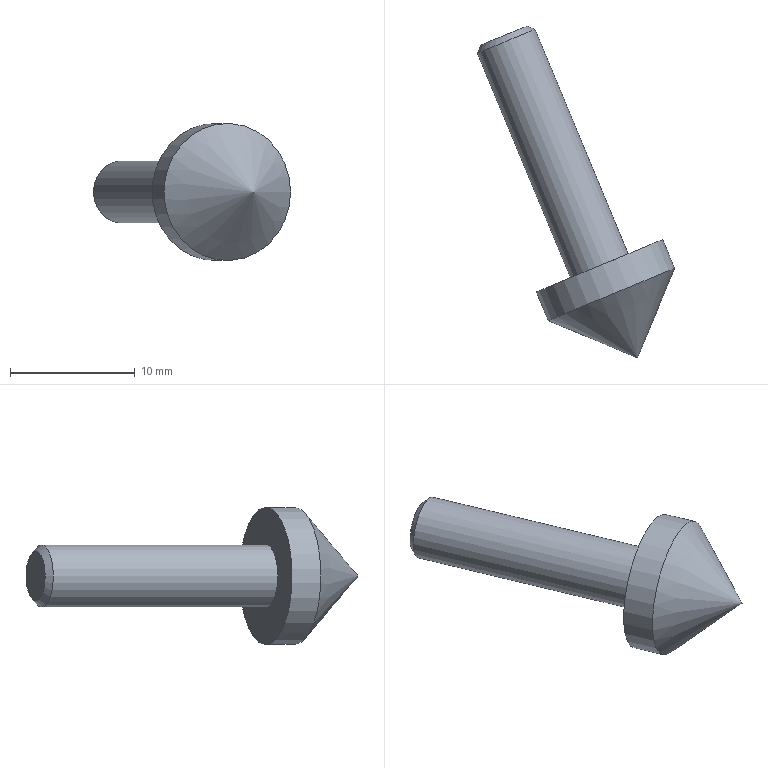Component | NX | PULLPIN | 1 solid | 6 faces | box 15.82 x 26.63 x 11 mm | volume 803 mm3 | plane 2 | cylinder 2 | cone 2 | commonest cylinder face diameters 5 x1 11 x1
STEP:
#1=CARTESIAN_POINT('',(0.,0.,0.));
#2=DIRECTION('',(0.,0.,1.));
#3=DIRECTION('',(1.,0.,0.));
#4=AXIS2_PLACEMENT_3D('',#1,#2,#3);
#5=CARTESIAN_POINT('',(-32.253,91.847,320.473));
#6=VERTEX_POINT('',#5);
#7=CARTESIAN_POINT('',(-30.405,92.613,320.473));
#8=DIRECTION('',(-0.383,0.9237,0.));
#9=DIRECTION('',(-0.9237,-0.383,0.));
#10=AXIS2_PLACEMENT_3D('',#7,#8,#9);
#11=CIRCLE('',#10,2.);
#12=CARTESIAN_POINT('',(-28.096,93.571,320.473));
#13=DIRECTION('',(0.383,-0.9237,0.));
#14=DIRECTION('',(-0.9237,-0.383,0.));
#15=AXIS2_PLACEMENT_3D('',#12,#13,#14);
#16=PLANE('',#15);
#17=CARTESIAN_POINT('',(4.5,0.));
#18=CARTESIAN_POINT('',(4.5,-3.464));
#19=CARTESIAN_POINT('',(1.5,-1.732));
#20=CARTESIAN_POINT('',(-1.5,-0.));
#21=CARTESIAN_POINT('',(1.5,1.732));
#22=CARTESIAN_POINT('',(4.5,3.464));
#23=CARTESIAN_POINT('',(4.5,0.));
#24=(BOUNDED_CURVE()B_SPLINE_CURVE(2,(#17,#18,#19,#20,#21,#22,#23),.UNSPECIFIED.,.T.,.F.)B_SPLINE_CURVE_WITH_KNOTS((1,2,2,2,2,1),(-2.094,0.,2.094,4.189,6.283,8.378),.UNSPECIFIED.)CURVE()GEOMETRIC_REPRESENTATION_ITEM()RATIONAL_B_SPLINE_CURVE((1.,0.5,1.,0.5,1.,0.5,1.))REPRESENTATION_ITEM(''));
#25=(GEOMETRIC_REPRESENTATION_CONTEXT(2)PARAMETRIC_REPRESENTATION_CONTEXT()REPRESENTATION_CONTEXT('',''));
#26=DEFINITIONAL_REPRESENTATION('',(#24),#25);
#27=PCURVE('',#16,#26);
#28=CARTESIAN_POINT('',(-30.405,92.613,320.473));
#29=DIRECTION('',(0.383,-0.9237,0.));
#30=DIRECTION('',(-0.9237,-0.383,0.));
#31=AXIS2_PLACEMENT_3D('',#28,#29,#30);
#32=CONICAL_SURFACE('',#31,2.,0.7854);
#33=CARTESIAN_POINT('',(6.283,0.));
#34=DIRECTION('',(-1.,0.));
#35=VECTOR('',#34,1.);
#36=LINE('',#33,#35);
#37=(GEOMETRIC_REPRESENTATION_CONTEXT(2)PARAMETRIC_REPRESENTATION_CONTEXT()REPRESENTATION_CONTEXT('',''));
#38=DEFINITIONAL_REPRESENTATION('',(#36),#37);
#39=PCURVE('',#32,#38);
#40=SURFACE_CURVE('',#11,(#27,#39),.PCURVE_S1.);
#41=EDGE_CURVE('',#6,#6,#40,.T.);
#42=ORIENTED_EDGE('',*,*,#41,.T.);
#43=EDGE_LOOP('',(#42));
#44=FACE_BOUND('',#43,.T.);
#45=ADVANCED_FACE('',(#44),#16,.F.);
#46=CARTESIAN_POINT('',(-32.523,91.194,320.473));
#47=VERTEX_POINT('',#46);
#48=CARTESIAN_POINT('',(-27.904,93.109,320.473));
#49=VERTEX_POINT('',#48);
#50=CARTESIAN_POINT('',(-30.214,92.152,320.473));
#51=DIRECTION('',(0.383,-0.9237,0.));
#52=DIRECTION('',(-0.9237,-0.383,0.));
#53=AXIS2_PLACEMENT_3D('',#50,#51,#52);
#54=CIRCLE('',#53,2.5);
#55=CARTESIAN_POINT('',(-19.68,66.749,320.473));
#56=DIRECTION('',(-0.383,0.9237,0.));
#57=DIRECTION('',(0.9237,0.383,0.));
#58=AXIS2_PLACEMENT_3D('',#55,#56,#57);
#59=CYLINDRICAL_SURFACE('',#58,2.5);
#60=CARTESIAN_POINT('',(3.142,27.5));
#61=DIRECTION('',(-1.,0.));
#62=VECTOR('',#61,1.);
#63=LINE('',#60,#62);
#64=(GEOMETRIC_REPRESENTATION_CONTEXT(2)PARAMETRIC_REPRESENTATION_CONTEXT()REPRESENTATION_CONTEXT('',''));
#65=DEFINITIONAL_REPRESENTATION('',(#63),#64);
#66=PCURVE('',#59,#65);
#67=CARTESIAN_POINT('',(0.,0.5));
#68=DIRECTION('',(1.,-0.));
#69=VECTOR('',#68,1.);
#70=LINE('',#67,#69);
#71=(GEOMETRIC_REPRESENTATION_CONTEXT(2)PARAMETRIC_REPRESENTATION_CONTEXT()REPRESENTATION_CONTEXT('',''));
#72=DEFINITIONAL_REPRESENTATION('',(#70),#71);
#73=PCURVE('',#32,#72);
#74=SURFACE_CURVE('',#54,(#66,#73),.PCURVE_S1.);
#75=EDGE_CURVE('',#47,#49,#74,.T.);
#76=ORIENTED_EDGE('',*,*,#75,.T.);
#77=CARTESIAN_POINT('',(-20.435,75.096,320.473));
#78=VERTEX_POINT('',#77);
#79=CARTESIAN_POINT('',(-20.435,75.096,320.473));
#80=CARTESIAN_POINT('',(-27.904,93.109,320.473));
#81=B_SPLINE_CURVE_WITH_KNOTS('',1,(#79,#80),.UNSPECIFIED.,.F.,.F.,(2,2),(8.,27.5),.PIECEWISE_BEZIER_KNOTS.);
#82=CARTESIAN_POINT('',(0.,0.));
#83=DIRECTION('',(0.,1.));
#84=VECTOR('',#83,1.);
#85=LINE('',#82,#84);
#86=(GEOMETRIC_REPRESENTATION_CONTEXT(2)PARAMETRIC_REPRESENTATION_CONTEXT()REPRESENTATION_CONTEXT('',''));
#87=DEFINITIONAL_REPRESENTATION('',(#85),#86);
#88=PCURVE('',#59,#87);
#89=CARTESIAN_POINT('',(6.283,0.));
#90=DIRECTION('',(0.,1.));
#91=VECTOR('',#90,1.);
#92=LINE('',#89,#91);
#93=(GEOMETRIC_REPRESENTATION_CONTEXT(2)PARAMETRIC_REPRESENTATION_CONTEXT()REPRESENTATION_CONTEXT('',''));
#94=DEFINITIONAL_REPRESENTATION('',(#92),#93);
#95=PCURVE('',#59,#94);
#96=SEAM_CURVE('',#81,(#88,#95),.PCURVE_S1.);
#97=EDGE_CURVE('',#78,#49,#96,.T.);
#98=ORIENTED_EDGE('',*,*,#97,.F.);
#99=CARTESIAN_POINT('',(-22.744,74.139,320.473));
#100=DIRECTION('',(-0.383,0.9237,0.));
#101=DIRECTION('',(0.9237,0.383,0.));
#102=AXIS2_PLACEMENT_3D('',#99,#100,#101);
#103=CIRCLE('',#102,2.5);
#104=CARTESIAN_POINT('',(0.,8.));
#105=DIRECTION('',(1.,0.));
#106=VECTOR('',#105,1.);
#107=LINE('',#104,#106);
#108=(GEOMETRIC_REPRESENTATION_CONTEXT(2)PARAMETRIC_REPRESENTATION_CONTEXT()REPRESENTATION_CONTEXT('',''));
#109=DEFINITIONAL_REPRESENTATION('',(#107),#108);
#110=PCURVE('',#59,#109);
#111=CARTESIAN_POINT('',(-17.664,76.246,320.473));
#112=DIRECTION('',(0.383,-0.9237,0.));
#113=DIRECTION('',(-0.9237,-0.383,0.));
#114=AXIS2_PLACEMENT_3D('',#111,#112,#113);
#115=PLANE('',#114);
#116=CARTESIAN_POINT('',(3.,0.));
#117=CARTESIAN_POINT('',(3.,4.33));
#118=CARTESIAN_POINT('',(6.75,2.165));
#119=CARTESIAN_POINT('',(10.5,0.));
#120=CARTESIAN_POINT('',(6.75,-2.165));
#121=CARTESIAN_POINT('',(3.,-4.33));
#122=CARTESIAN_POINT('',(3.,0.));
#123=(BOUNDED_CURVE()B_SPLINE_CURVE(2,(#116,#117,#118,#119,#120,#121,#122),.UNSPECIFIED.,.T.,.F.)B_SPLINE_CURVE_WITH_KNOTS((1,2,2,2,2,1),(-2.094,0.,2.094,4.189,6.283,8.378),.UNSPECIFIED.)CURVE()GEOMETRIC_REPRESENTATION_ITEM()RATIONAL_B_SPLINE_CURVE((1.,0.5,1.,0.5,1.,0.5,1.))REPRESENTATION_ITEM(''));
#124=(GEOMETRIC_REPRESENTATION_CONTEXT(2)PARAMETRIC_REPRESENTATION_CONTEXT()REPRESENTATION_CONTEXT('',''));
#125=DEFINITIONAL_REPRESENTATION('',(#123),#124);
#126=PCURVE('',#115,#125);
#127=SURFACE_CURVE('',#103,(#110,#126),.PCURVE_S1.);
#128=EDGE_CURVE('',#78,#78,#127,.T.);
#129=ORIENTED_EDGE('',*,*,#128,.T.);
#130=ORIENTED_EDGE('',*,*,#97,.T.);
#131=CARTESIAN_POINT('',(-30.214,92.152,320.473));
#132=DIRECTION('',(0.383,-0.9237,0.));
#133=DIRECTION('',(-0.9237,-0.383,0.));
#134=AXIS2_PLACEMENT_3D('',#131,#132,#133);
#135=CIRCLE('',#134,2.5);
#136=CARTESIAN_POINT('',(9.425,27.5));
#137=DIRECTION('',(-1.,0.));
#138=VECTOR('',#137,1.);
#139=LINE('',#136,#138);
#140=(GEOMETRIC_REPRESENTATION_CONTEXT(2)PARAMETRIC_REPRESENTATION_CONTEXT()REPRESENTATION_CONTEXT('',''));
#141=DEFINITIONAL_REPRESENTATION('',(#139),#140);
#142=PCURVE('',#59,#141);
#143=CARTESIAN_POINT('',(0.,0.5));
#144=DIRECTION('',(1.,0.));
#145=VECTOR('',#144,1.);
#146=LINE('',#143,#145);
#147=(GEOMETRIC_REPRESENTATION_CONTEXT(2)PARAMETRIC_REPRESENTATION_CONTEXT()REPRESENTATION_CONTEXT('',''));
#148=DEFINITIONAL_REPRESENTATION('',(#146),#147);
#149=PCURVE('',#32,#148);
#150=SURFACE_CURVE('',#135,(#142,#149),.PCURVE_S1.);
#151=EDGE_CURVE('',#49,#47,#150,.T.);
#152=ORIENTED_EDGE('',*,*,#151,.T.);
#153=EDGE_LOOP('',(#76,#98,#129,#130,#152));
#154=FACE_BOUND('',#153,.T.);
#155=ADVANCED_FACE('',(#154),#59,.T.);
#156=ORIENTED_EDGE('',*,*,#128,.F.);
#157=EDGE_LOOP('',(#156));
#158=FACE_BOUND('',#157,.T.);
#159=CARTESIAN_POINT('',(-17.664,76.246,320.473));
#160=VERTEX_POINT('',#159);
#161=CARTESIAN_POINT('',(-22.744,74.139,320.473));
#162=DIRECTION('',(-0.383,0.9237,0.));
#163=DIRECTION('',(0.9237,0.383,0.));
#164=AXIS2_PLACEMENT_3D('',#161,#162,#163);
#165=CIRCLE('',#164,5.5);
#166=CARTESIAN_POINT('',(0.,0.));
#167=CARTESIAN_POINT('',(0.,9.526));
#168=CARTESIAN_POINT('',(8.25,4.763));
#169=CARTESIAN_POINT('',(16.5,0.));
#170=CARTESIAN_POINT('',(8.25,-4.763));
#171=CARTESIAN_POINT('',(0.,-9.526));
#172=CARTESIAN_POINT('',(0.,0.));
#173=(BOUNDED_CURVE()B_SPLINE_CURVE(2,(#166,#167,#168,#169,#170,#171,#172),.UNSPECIFIED.,.T.,.F.)B_SPLINE_CURVE_WITH_KNOTS((1,2,2,2,2,1),(-2.094,0.,2.094,4.189,6.283,8.378),.UNSPECIFIED.)CURVE()GEOMETRIC_REPRESENTATION_ITEM()RATIONAL_B_SPLINE_CURVE((1.,0.5,1.,0.5,1.,0.5,1.))REPRESENTATION_ITEM(''));
#174=(GEOMETRIC_REPRESENTATION_CONTEXT(2)PARAMETRIC_REPRESENTATION_CONTEXT()REPRESENTATION_CONTEXT('',''));
#175=DEFINITIONAL_REPRESENTATION('',(#173),#174);
#176=PCURVE('',#115,#175);
#177=CARTESIAN_POINT('',(-19.68,66.749,320.473));
#178=DIRECTION('',(-0.383,0.9237,0.));
#179=DIRECTION('',(0.9237,0.383,0.));
#180=AXIS2_PLACEMENT_3D('',#177,#178,#179);
#181=CYLINDRICAL_SURFACE('',#180,5.5);
#182=CARTESIAN_POINT('',(0.,8.));
#183=DIRECTION('',(1.,0.));
#184=VECTOR('',#183,1.);
#185=LINE('',#182,#184);
#186=(GEOMETRIC_REPRESENTATION_CONTEXT(2)PARAMETRIC_REPRESENTATION_CONTEXT()REPRESENTATION_CONTEXT('',''));
#187=DEFINITIONAL_REPRESENTATION('',(#185),#186);
#188=PCURVE('',#181,#187);
#189=SURFACE_CURVE('',#165,(#176,#188),.PCURVE_S1.);
#190=EDGE_CURVE('',#160,#160,#189,.T.);
#191=ORIENTED_EDGE('',*,*,#190,.T.);
#192=EDGE_LOOP('',(#191));
#193=FACE_BOUND('',#192,.T.);
#194=ADVANCED_FACE('',(#158,#193),#115,.F.);
#195=ORIENTED_EDGE('',*,*,#190,.F.);
#196=CARTESIAN_POINT('',(-16.706,73.936,320.473));
#197=VERTEX_POINT('',#196);
#198=CARTESIAN_POINT('',(-16.706,73.936,320.473));
#199=CARTESIAN_POINT('',(-17.664,76.246,320.473));
#200=B_SPLINE_CURVE_WITH_KNOTS('',1,(#198,#199),.UNSPECIFIED.,.F.,.F.,(2,2),(5.5,8.),.PIECEWISE_BEZIER_KNOTS.);
#201=CARTESIAN_POINT('',(0.,0.));
#202=DIRECTION('',(0.,1.));
#203=VECTOR('',#202,1.);
#204=LINE('',#201,#203);
#205=(GEOMETRIC_REPRESENTATION_CONTEXT(2)PARAMETRIC_REPRESENTATION_CONTEXT()REPRESENTATION_CONTEXT('',''));
#206=DEFINITIONAL_REPRESENTATION('',(#204),#205);
#207=PCURVE('',#181,#206);
#208=CARTESIAN_POINT('',(6.283,0.));
#209=DIRECTION('',(0.,1.));
#210=VECTOR('',#209,1.);
#211=LINE('',#208,#210);
#212=(GEOMETRIC_REPRESENTATION_CONTEXT(2)PARAMETRIC_REPRESENTATION_CONTEXT()REPRESENTATION_CONTEXT('',''));
#213=DEFINITIONAL_REPRESENTATION('',(#211),#212);
#214=PCURVE('',#181,#213);
#215=SEAM_CURVE('',#200,(#207,#214),.PCURVE_S1.);
#216=EDGE_CURVE('',#197,#160,#215,.T.);
#217=ORIENTED_EDGE('',*,*,#216,.F.);
#218=CARTESIAN_POINT('',(-21.787,71.829,320.473));
#219=DIRECTION('',(-0.383,0.9237,0.));
#220=DIRECTION('',(0.9237,0.383,0.));
#221=AXIS2_PLACEMENT_3D('',#218,#219,#220);
#222=CIRCLE('',#221,5.5);
#223=CARTESIAN_POINT('',(0.,5.5));
#224=DIRECTION('',(1.,0.));
#225=VECTOR('',#224,1.);
#226=LINE('',#223,#225);
#227=(GEOMETRIC_REPRESENTATION_CONTEXT(2)PARAMETRIC_REPRESENTATION_CONTEXT()REPRESENTATION_CONTEXT('',''));
#228=DEFINITIONAL_REPRESENTATION('',(#226),#227);
#229=PCURVE('',#181,#228);
#230=CARTESIAN_POINT('',(-19.68,66.749,320.473));
#231=DIRECTION('',(-0.383,0.9237,0.));
#232=DIRECTION('',(0.9237,0.383,0.));
#233=AXIS2_PLACEMENT_3D('',#230,#231,#232);
#234=CONICAL_SURFACE('',#233,0.,0.7854);
#235=CARTESIAN_POINT('',(0.,5.5));
#236=DIRECTION('',(1.,0.));
#237=VECTOR('',#236,1.);
#238=LINE('',#235,#237);
#239=(GEOMETRIC_REPRESENTATION_CONTEXT(2)PARAMETRIC_REPRESENTATION_CONTEXT()REPRESENTATION_CONTEXT('',''));
#240=DEFINITIONAL_REPRESENTATION('',(#238),#239);
#241=PCURVE('',#234,#240);
#242=SURFACE_CURVE('',#222,(#229,#241),.PCURVE_S1.);
#243=EDGE_CURVE('',#197,#197,#242,.T.);
#244=ORIENTED_EDGE('',*,*,#243,.T.);
#245=ORIENTED_EDGE('',*,*,#216,.T.);
#246=EDGE_LOOP('',(#195,#217,#244,#245));
#247=FACE_BOUND('',#246,.T.);
#248=ADVANCED_FACE('',(#247),#181,.T.);
#249=ORIENTED_EDGE('',*,*,#243,.F.);
#250=CARTESIAN_POINT('',(-19.68,66.749,320.473));
#251=VERTEX_POINT('',#250);
#252=CARTESIAN_POINT('',(-19.68,66.749,320.473));
#253=CARTESIAN_POINT('',(-16.706,73.936,320.473));
#254=B_SPLINE_CURVE_WITH_KNOTS('',1,(#252,#253),.UNSPECIFIED.,.F.,.F.,(2,2),(0.,7.778),.PIECEWISE_BEZIER_KNOTS.);
#255=CARTESIAN_POINT('',(0.,0.));
#256=DIRECTION('',(0.,1.));
#257=VECTOR('',#256,1.);
#258=LINE('',#255,#257);
#259=(GEOMETRIC_REPRESENTATION_CONTEXT(2)PARAMETRIC_REPRESENTATION_CONTEXT()REPRESENTATION_CONTEXT('',''));
#260=DEFINITIONAL_REPRESENTATION('',(#258),#259);
#261=PCURVE('',#234,#260);
#262=CARTESIAN_POINT('',(6.283,0.));
#263=DIRECTION('',(0.,1.));
#264=VECTOR('',#263,1.);
#265=LINE('',#262,#264);
#266=(GEOMETRIC_REPRESENTATION_CONTEXT(2)PARAMETRIC_REPRESENTATION_CONTEXT()REPRESENTATION_CONTEXT('',''));
#267=DEFINITIONAL_REPRESENTATION('',(#265),#266);
#268=PCURVE('',#234,#267);
#269=SEAM_CURVE('',#254,(#261,#268),.PCURVE_S1.);
#270=EDGE_CURVE('',#251,#197,#269,.T.);
#271=ORIENTED_EDGE('',*,*,#270,.F.);
#272=ORIENTED_EDGE('',*,*,#270,.T.);
#273=EDGE_LOOP('',(#249,#271,#272));
#274=FACE_BOUND('',#273,.T.);
#275=ADVANCED_FACE('',(#274),#234,.T.);
#276=ORIENTED_EDGE('',*,*,#75,.F.);
#277=CARTESIAN_POINT('',(-32.253,91.847,320.473));
#278=CARTESIAN_POINT('',(-32.523,91.194,320.473));
#279=B_SPLINE_CURVE_WITH_KNOTS('',1,(#277,#278),.UNSPECIFIED.,.F.,.F.,(2,2),(0.,0.7071),.PIECEWISE_BEZIER_KNOTS.);
#280=CARTESIAN_POINT('',(0.,0.));
#281=DIRECTION('',(0.,1.));
#282=VECTOR('',#281,1.);
#283=LINE('',#280,#282);
#284=(GEOMETRIC_REPRESENTATION_CONTEXT(2)PARAMETRIC_REPRESENTATION_CONTEXT()REPRESENTATION_CONTEXT('',''));
#285=DEFINITIONAL_REPRESENTATION('',(#283),#284);
#286=PCURVE('',#32,#285);
#287=CARTESIAN_POINT('',(6.283,0.));
#288=DIRECTION('',(0.,1.));
#289=VECTOR('',#288,1.);
#290=LINE('',#287,#289);
#291=(GEOMETRIC_REPRESENTATION_CONTEXT(2)PARAMETRIC_REPRESENTATION_CONTEXT()REPRESENTATION_CONTEXT('',''));
#292=DEFINITIONAL_REPRESENTATION('',(#290),#291);
#293=PCURVE('',#32,#292);
#294=SEAM_CURVE('',#279,(#286,#293),.PCURVE_S1.);
#295=EDGE_CURVE('',#6,#47,#294,.T.);
#296=ORIENTED_EDGE('',*,*,#295,.F.);
#297=ORIENTED_EDGE('',*,*,#41,.F.);
#298=ORIENTED_EDGE('',*,*,#295,.T.);
#299=ORIENTED_EDGE('',*,*,#151,.F.);
#300=EDGE_LOOP('',(#276,#296,#297,#298,#299));
#301=FACE_BOUND('',#300,.T.);
#302=ADVANCED_FACE('',(#301),#32,.T.);
#303=CLOSED_SHELL('',(#45,#155,#194,#248,#275,#302));
#304=MANIFOLD_SOLID_BREP('',#303);
#305=(LENGTH_UNIT()NAMED_UNIT(*)SI_UNIT(.MILLI.,.METRE.));
#306=UNCERTAINTY_MEASURE_WITH_UNIT(LENGTH_MEASURE(0.00001),#305,'','');
#307=(NAMED_UNIT(*)PLANE_ANGLE_UNIT()SI_UNIT($,.RADIAN.));
#308=(NAMED_UNIT(*)SI_UNIT($,.STERADIAN.)SOLID_ANGLE_UNIT());
#309=(GEOMETRIC_REPRESENTATION_CONTEXT(3)GLOBAL_UNCERTAINTY_ASSIGNED_CONTEXT((#306))GLOBAL_UNIT_ASSIGNED_CONTEXT((#305,#307,#308))REPRESENTATION_CONTEXT('',''));
#310=ADVANCED_BREP_SHAPE_REPRESENTATION('',(#4,#304),#309);